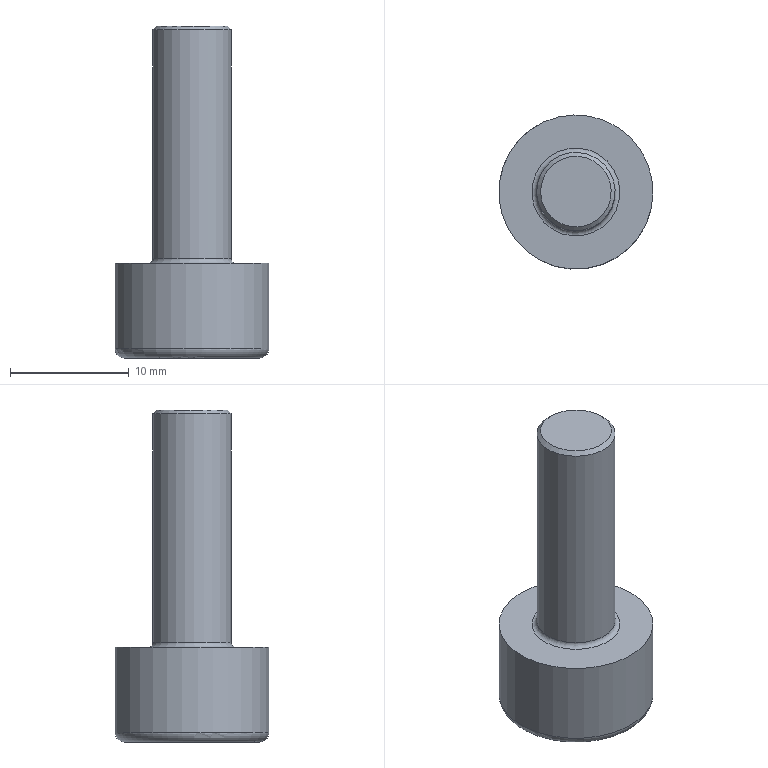Component | NX | SCREW_M8X20 | 1 solid | 27 faces | volume 1580 mm3 | plane 15 | cone 8 | cylinder 2 | torus 2 | commonest cylinder face diameters 6.619 x1 13 x1